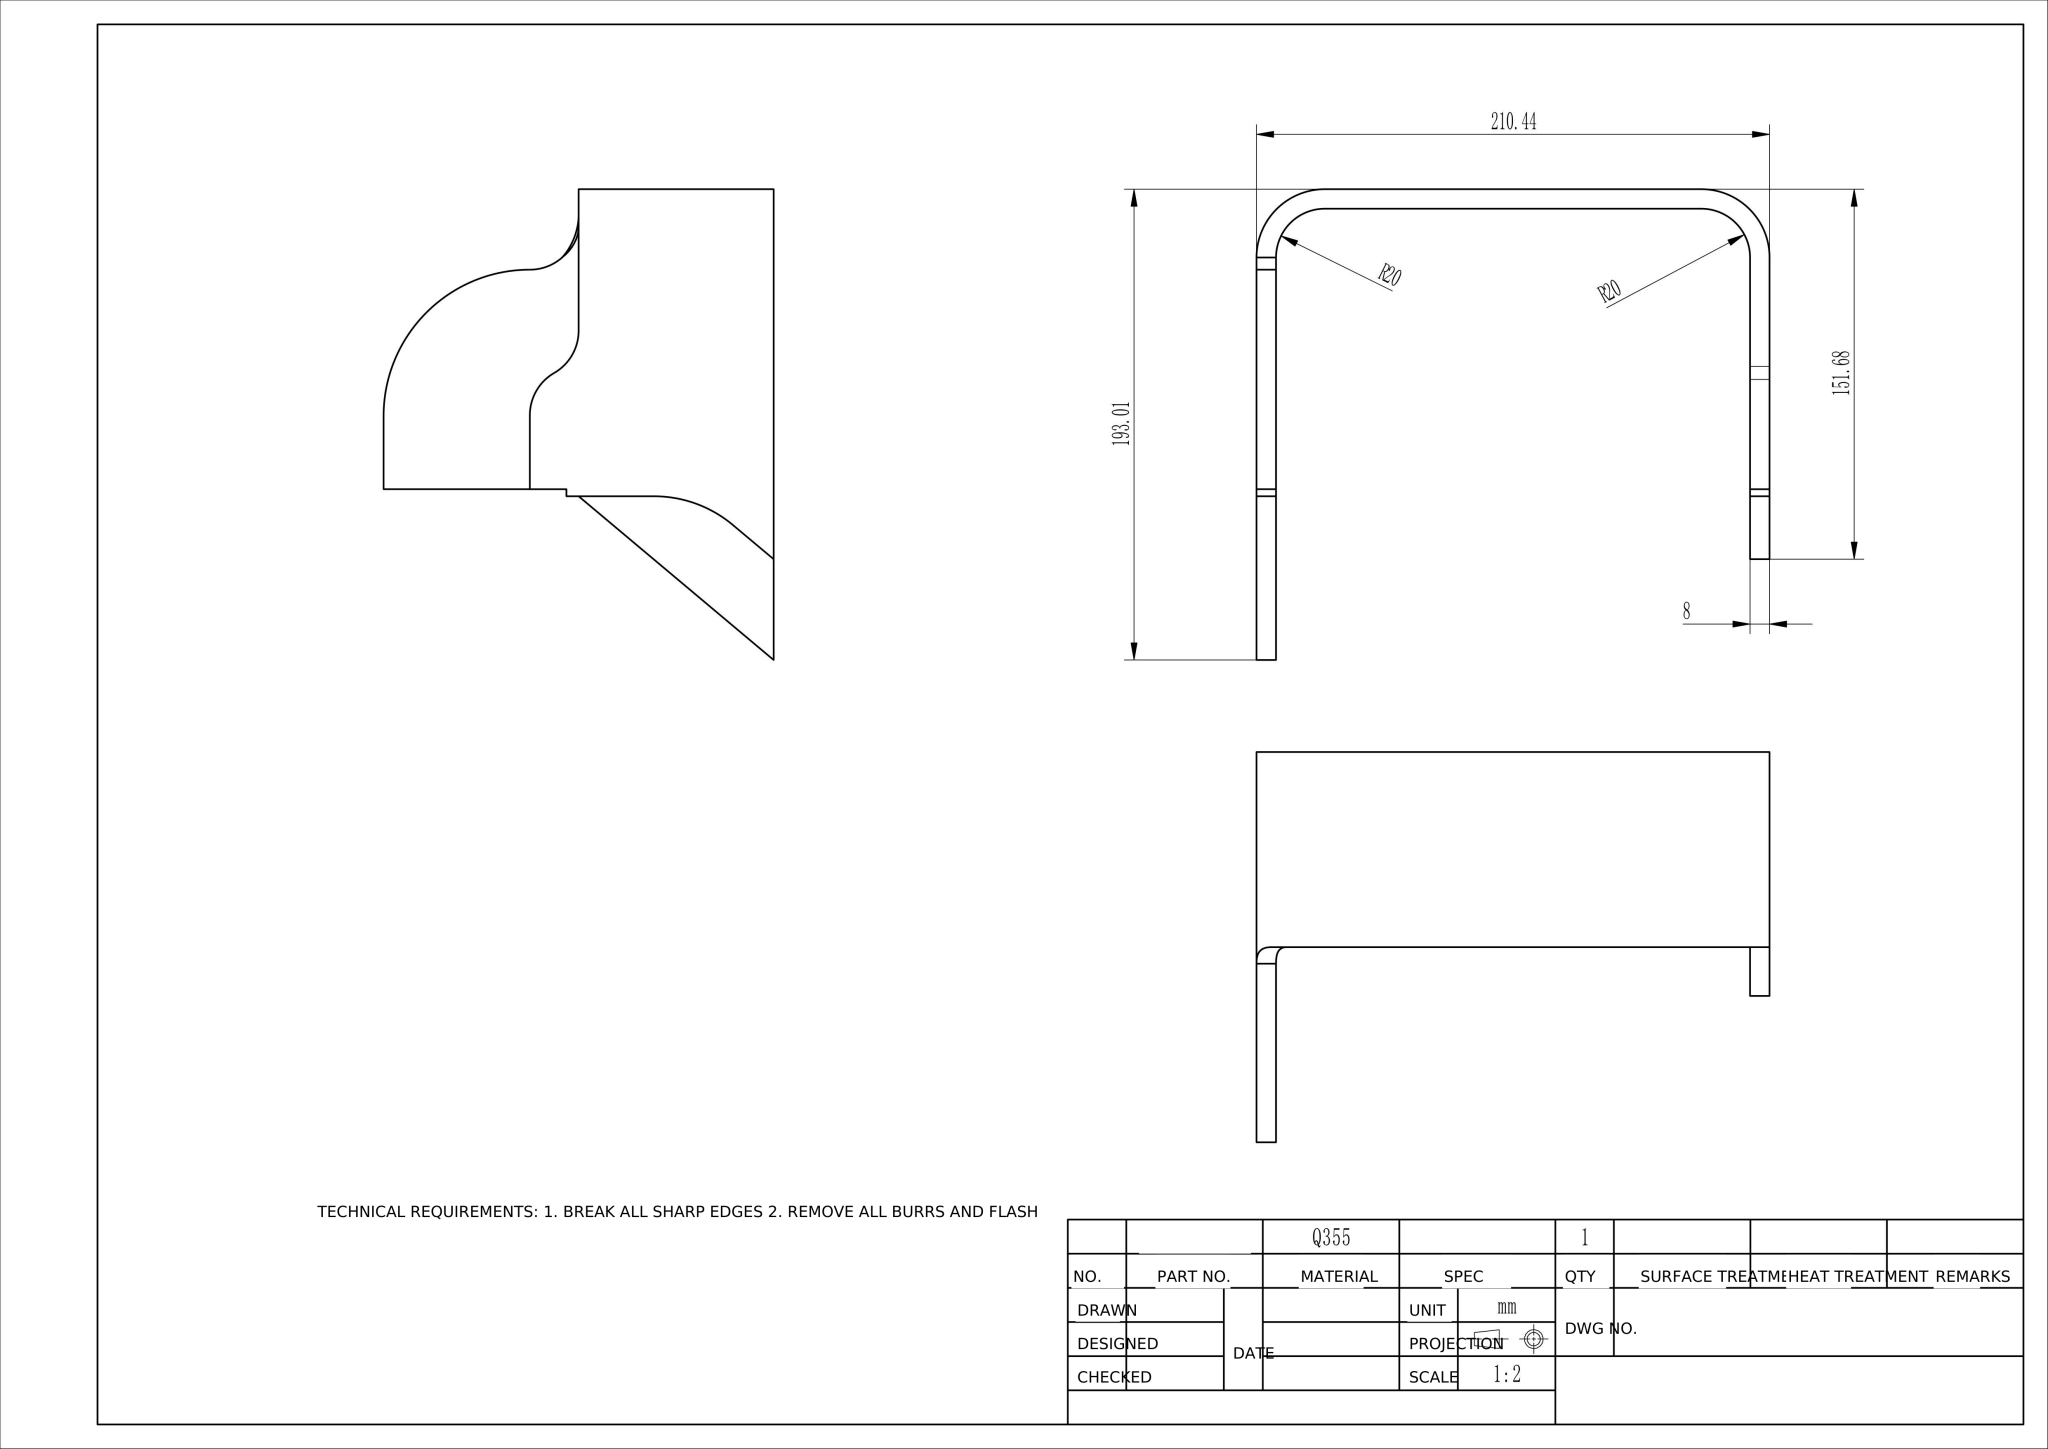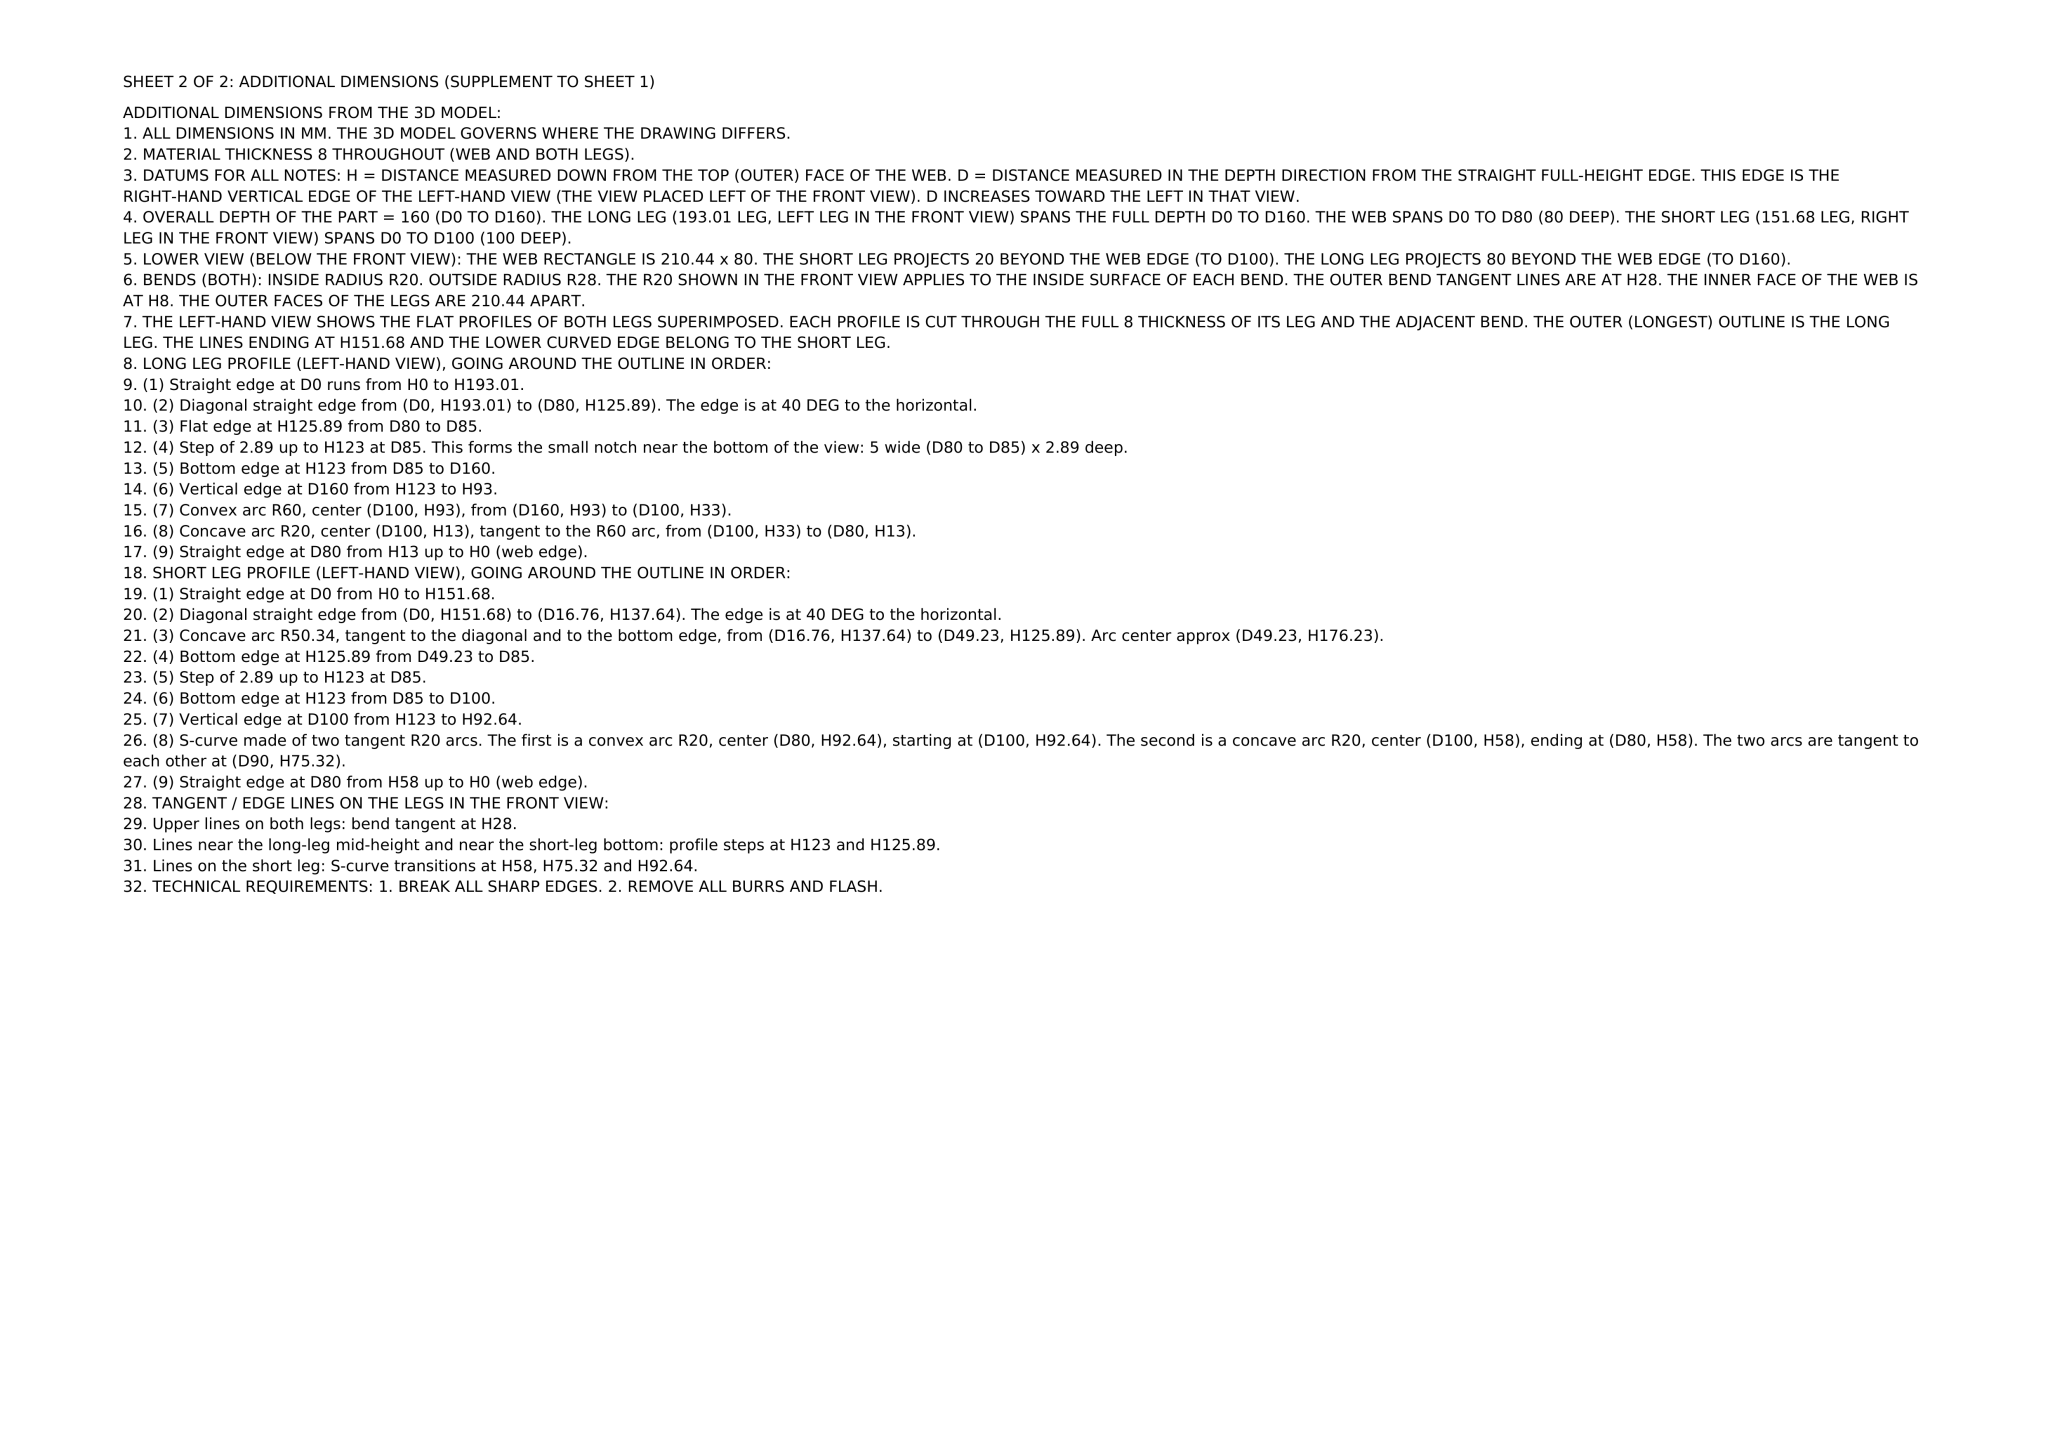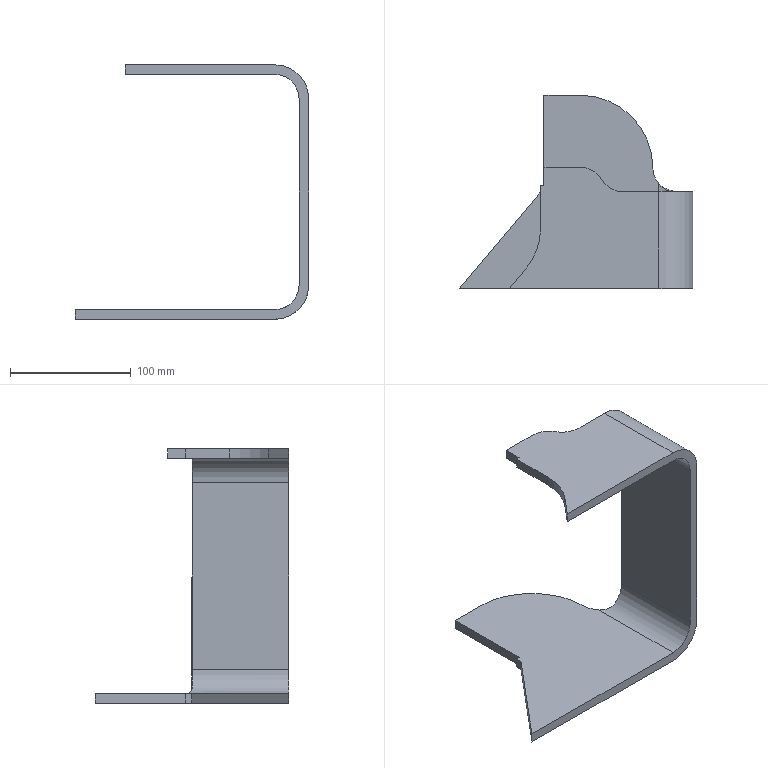Part | NX | mm | 1 solid | 28 faces | box 193.01 x 160 x 210.44 mm | volume 357331 mm3 | plane 18 | cylinder 9 | spline 1 | commonest cylinder face diameters 40 x5 56 x2 120 x1 100.67 x1